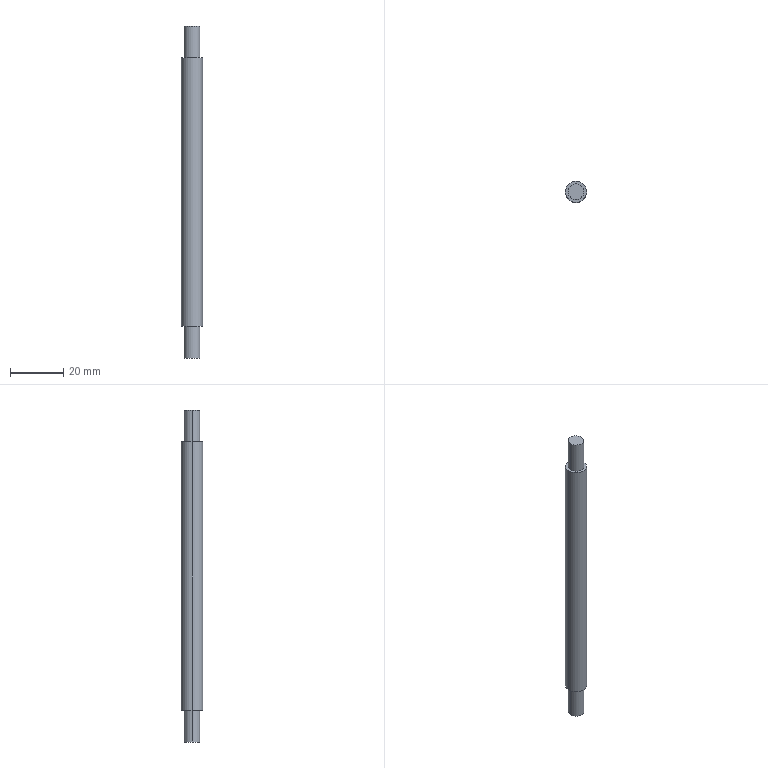Component | SolidWorks | TAR-02-024PaperPressWheelAxis-1 | 1 solid | 10 faces | box 8 x 8 x 125 mm | volume 5755 mm3 | cylinder 6 | plane 4 | commonest cylinder face diameters 6 x4 8 x2
build123d program:
from build123d import *

# Parameters (mm, degrees)
SKETCH1_R           = 3
BOSS_EXTRUDE1_DEPTH = 12
SKETCH2_R           = 4
BOSS_EXTRUDE2_DEPTH = 101


with BuildPart() as part:
    # Sketch1 → Boss-Extrude1 (new body)
    with BuildSketch(Plane.XY):
        Circle(SKETCH1_R)
    boss_extrude1 = extrude(amount=BOSS_EXTRUDE1_DEPTH)

    # Sketch2 → Boss-Extrude2 (add)
    with BuildSketch(Plane.XY.offset(12)):
        Circle(SKETCH2_R)
    extrude(amount=BOSS_EXTRUDE2_DEPTH)

    # Mirror1: Boss-Extrude1 across plane
    add(boss_extrude1.mirror(Plane(origin=(0, 0, 62.5), x_dir=(1, 0, 0), z_dir=(0, 0, -1))))


solid = part.part

# Placed as in the assembly
solid = solid.moved(Location((8.333, 43.101, -156.165), (0, 0, 0)))
STEP:
#1=CARTESIAN_POINT('',(0.4462,1.697,-1.699));
#2=VERTEX_POINT('',#1);
#3=CARTESIAN_POINT('',(0.2099,1.697,-1.699));
#4=VERTEX_POINT('',#3);
#5=CARTESIAN_POINT('',(0.3281,1.697,-1.699));
#6=DIRECTION('',(0.,0.,1.));
#7=DIRECTION('',(1.,0.,0.));
#8=AXIS2_PLACEMENT_3D('',#5,#6,#7);
#9=CIRCLE('',#8,0.1181);
#10=EDGE_CURVE('',#2,#4,#9,.T.);
#11=ORIENTED_EDGE('',*,*,#10,.T.);
#12=CARTESIAN_POINT('',(0.2099,1.697,-1.227));
#13=VERTEX_POINT('',#12);
#14=CARTESIAN_POINT('',(0.2099,1.697,-1.699));
#15=DIRECTION('',(0.,0.,1.));
#16=VECTOR('',#15,39.37);
#17=LINE('',#14,#16);
#18=EDGE_CURVE('',#4,#13,#17,.T.);
#19=ORIENTED_EDGE('',*,*,#18,.T.);
#20=CARTESIAN_POINT('',(0.4462,1.697,-1.227));
#21=VERTEX_POINT('',#20);
#22=CARTESIAN_POINT('',(0.3281,1.697,-1.227));
#23=DIRECTION('',(0.,0.,1.));
#24=DIRECTION('',(1.,0.,0.));
#25=AXIS2_PLACEMENT_3D('',#22,#23,#24);
#26=CIRCLE('',#25,0.1181);
#27=EDGE_CURVE('',#21,#13,#26,.T.);
#28=ORIENTED_EDGE('',*,*,#27,.F.);
#29=CARTESIAN_POINT('',(0.4462,1.697,-1.699));
#30=DIRECTION('',(0.,0.,1.));
#31=VECTOR('',#30,39.37);
#32=LINE('',#29,#31);
#33=EDGE_CURVE('',#2,#21,#32,.T.);
#34=ORIENTED_EDGE('',*,*,#33,.F.);
#35=EDGE_LOOP('',(#11,#19,#28,#34));
#36=FACE_OUTER_BOUND('',#35,.T.);
#37=CARTESIAN_POINT('',(0.3281,1.697,-1.699));
#38=DIRECTION('',(0.,0.,1.));
#39=DIRECTION('',(1.,0.,0.));
#40=AXIS2_PLACEMENT_3D('',#37,#38,#39);
#41=CYLINDRICAL_SURFACE('',#40,0.1181);
#42=ADVANCED_FACE('',(#36),#41,.T.);
#43=CARTESIAN_POINT('',(0.4855,1.697,-1.699));
#44=VERTEX_POINT('',#43);
#45=CARTESIAN_POINT('',(0.1706,1.697,-1.699));
#46=VERTEX_POINT('',#45);
#47=CARTESIAN_POINT('',(0.3281,1.697,-1.699));
#48=DIRECTION('',(0.,0.,1.));
#49=DIRECTION('',(1.,0.,0.));
#50=AXIS2_PLACEMENT_3D('',#47,#48,#49);
#51=CIRCLE('',#50,0.1575);
#52=EDGE_CURVE('',#44,#46,#51,.T.);
#53=ORIENTED_EDGE('',*,*,#52,.F.);
#54=CARTESIAN_POINT('',(0.4855,1.697,-5.676));
#55=VERTEX_POINT('',#54);
#56=CARTESIAN_POINT('',(0.4855,1.697,-1.699));
#57=DIRECTION('',(0.,0.,-1.));
#58=VECTOR('',#57,39.37);
#59=LINE('',#56,#58);
#60=EDGE_CURVE('',#44,#55,#59,.T.);
#61=ORIENTED_EDGE('',*,*,#60,.T.);
#62=CARTESIAN_POINT('',(0.1706,1.697,-5.676));
#63=VERTEX_POINT('',#62);
#64=CARTESIAN_POINT('',(0.3281,1.697,-5.676));
#65=DIRECTION('',(0.,0.,1.));
#66=DIRECTION('',(1.,0.,0.));
#67=AXIS2_PLACEMENT_3D('',#64,#65,#66);
#68=CIRCLE('',#67,0.1575);
#69=EDGE_CURVE('',#55,#63,#68,.T.);
#70=ORIENTED_EDGE('',*,*,#69,.T.);
#71=CARTESIAN_POINT('',(0.1706,1.697,-1.699));
#72=DIRECTION('',(0.,0.,-1.));
#73=VECTOR('',#72,39.37);
#74=LINE('',#71,#73);
#75=EDGE_CURVE('',#46,#63,#74,.T.);
#76=ORIENTED_EDGE('',*,*,#75,.F.);
#77=EDGE_LOOP('',(#53,#61,#70,#76));
#78=FACE_OUTER_BOUND('',#77,.T.);
#79=CARTESIAN_POINT('',(0.3281,1.697,-1.699));
#80=DIRECTION('',(0.,0.,-1.));
#81=DIRECTION('',(-1.,0.,0.));
#82=AXIS2_PLACEMENT_3D('',#79,#80,#81);
#83=CYLINDRICAL_SURFACE('',#82,0.1575);
#84=ADVANCED_FACE('',(#78),#83,.T.);
#85=CARTESIAN_POINT('',(0.4462,1.697,-5.676));
#86=VERTEX_POINT('',#85);
#87=CARTESIAN_POINT('',(0.2099,1.697,-5.676));
#88=VERTEX_POINT('',#87);
#89=CARTESIAN_POINT('',(0.3281,1.697,-5.676));
#90=DIRECTION('',(0.,0.,1.));
#91=DIRECTION('',(1.,0.,0.));
#92=AXIS2_PLACEMENT_3D('',#89,#90,#91);
#93=CIRCLE('',#92,0.1181);
#94=EDGE_CURVE('',#86,#88,#93,.T.);
#95=ORIENTED_EDGE('',*,*,#94,.F.);
#96=CARTESIAN_POINT('',(0.4462,1.697,-6.148));
#97=VERTEX_POINT('',#96);
#98=CARTESIAN_POINT('',(0.4462,1.697,-5.676));
#99=DIRECTION('',(0.,0.,-1.));
#100=VECTOR('',#99,39.37);
#101=LINE('',#98,#100);
#102=EDGE_CURVE('',#86,#97,#101,.T.);
#103=ORIENTED_EDGE('',*,*,#102,.T.);
#104=CARTESIAN_POINT('',(0.2099,1.697,-6.148));
#105=VERTEX_POINT('',#104);
#106=CARTESIAN_POINT('',(0.3281,1.697,-6.148));
#107=DIRECTION('',(0.,0.,1.));
#108=DIRECTION('',(1.,0.,0.));
#109=AXIS2_PLACEMENT_3D('',#106,#107,#108);
#110=CIRCLE('',#109,0.1181);
#111=EDGE_CURVE('',#97,#105,#110,.T.);
#112=ORIENTED_EDGE('',*,*,#111,.T.);
#113=CARTESIAN_POINT('',(0.2099,1.697,-5.676));
#114=DIRECTION('',(0.,0.,-1.));
#115=VECTOR('',#114,39.37);
#116=LINE('',#113,#115);
#117=EDGE_CURVE('',#88,#105,#116,.T.);
#118=ORIENTED_EDGE('',*,*,#117,.F.);
#119=EDGE_LOOP('',(#95,#103,#112,#118));
#120=FACE_OUTER_BOUND('',#119,.T.);
#121=CARTESIAN_POINT('',(0.3281,1.697,-5.676));
#122=DIRECTION('',(0.,0.,-1.));
#123=DIRECTION('',(-1.,0.,0.));
#124=AXIS2_PLACEMENT_3D('',#121,#122,#123);
#125=CYLINDRICAL_SURFACE('',#124,0.1181);
#126=ADVANCED_FACE('',(#120),#125,.T.);
#127=ORIENTED_EDGE('',*,*,#102,.F.);
#128=CARTESIAN_POINT('',(0.3281,1.697,-5.676));
#129=DIRECTION('',(0.,0.,1.));
#130=DIRECTION('',(1.,0.,0.));
#131=AXIS2_PLACEMENT_3D('',#128,#129,#130);
#132=CIRCLE('',#131,0.1181);
#133=EDGE_CURVE('',#88,#86,#132,.T.);
#134=ORIENTED_EDGE('',*,*,#133,.F.);
#135=ORIENTED_EDGE('',*,*,#117,.T.);
#136=CARTESIAN_POINT('',(0.3281,1.697,-6.148));
#137=DIRECTION('',(0.,0.,1.));
#138=DIRECTION('',(1.,0.,0.));
#139=AXIS2_PLACEMENT_3D('',#136,#137,#138);
#140=CIRCLE('',#139,0.1181);
#141=EDGE_CURVE('',#105,#97,#140,.T.);
#142=ORIENTED_EDGE('',*,*,#141,.T.);
#143=EDGE_LOOP('',(#127,#134,#135,#142));
#144=FACE_OUTER_BOUND('',#143,.T.);
#145=CARTESIAN_POINT('',(0.3281,1.697,-5.676));
#146=DIRECTION('',(0.,0.,-1.));
#147=DIRECTION('',(-1.,0.,0.));
#148=AXIS2_PLACEMENT_3D('',#145,#146,#147);
#149=CYLINDRICAL_SURFACE('',#148,0.1181);
#150=ADVANCED_FACE('',(#144),#149,.T.);
#151=ORIENTED_EDGE('',*,*,#141,.F.);
#152=ORIENTED_EDGE('',*,*,#111,.F.);
#153=EDGE_LOOP('',(#151,#152));
#154=FACE_OUTER_BOUND('',#153,.T.);
#155=CARTESIAN_POINT('',(0.3281,1.697,-6.148));
#156=DIRECTION('',(0.,0.,1.));
#157=DIRECTION('',(1.,0.,0.));
#158=AXIS2_PLACEMENT_3D('',#155,#156,#157);
#159=PLANE('',#158);
#160=ADVANCED_FACE('',(#154),#159,.F.);
#161=ORIENTED_EDGE('',*,*,#60,.F.);
#162=CARTESIAN_POINT('',(0.3281,1.697,-1.699));
#163=DIRECTION('',(0.,0.,1.));
#164=DIRECTION('',(1.,0.,0.));
#165=AXIS2_PLACEMENT_3D('',#162,#163,#164);
#166=CIRCLE('',#165,0.1575);
#167=EDGE_CURVE('',#46,#44,#166,.T.);
#168=ORIENTED_EDGE('',*,*,#167,.F.);
#169=ORIENTED_EDGE('',*,*,#75,.T.);
#170=CARTESIAN_POINT('',(0.3281,1.697,-5.676));
#171=DIRECTION('',(0.,0.,1.));
#172=DIRECTION('',(1.,0.,0.));
#173=AXIS2_PLACEMENT_3D('',#170,#171,#172);
#174=CIRCLE('',#173,0.1575);
#175=EDGE_CURVE('',#63,#55,#174,.T.);
#176=ORIENTED_EDGE('',*,*,#175,.T.);
#177=EDGE_LOOP('',(#161,#168,#169,#176));
#178=FACE_OUTER_BOUND('',#177,.T.);
#179=CARTESIAN_POINT('',(0.3281,1.697,-1.699));
#180=DIRECTION('',(0.,0.,-1.));
#181=DIRECTION('',(-1.,0.,0.));
#182=AXIS2_PLACEMENT_3D('',#179,#180,#181);
#183=CYLINDRICAL_SURFACE('',#182,0.1575);
#184=ADVANCED_FACE('',(#178),#183,.T.);
#185=ORIENTED_EDGE('',*,*,#10,.F.);
#186=CARTESIAN_POINT('',(0.3281,1.697,-1.699));
#187=DIRECTION('',(0.,0.,1.));
#188=DIRECTION('',(1.,0.,0.));
#189=AXIS2_PLACEMENT_3D('',#186,#187,#188);
#190=CIRCLE('',#189,0.1181);
#191=EDGE_CURVE('',#4,#2,#190,.T.);
#192=ORIENTED_EDGE('',*,*,#191,.F.);
#193=EDGE_LOOP('',(#185,#192));
#194=FACE_BOUND('',#193,.T.);
#195=ORIENTED_EDGE('',*,*,#167,.T.);
#196=ORIENTED_EDGE('',*,*,#52,.T.);
#197=EDGE_LOOP('',(#195,#196));
#198=FACE_OUTER_BOUND('',#197,.T.);
#199=CARTESIAN_POINT('',(0.3281,1.697,-1.699));
#200=DIRECTION('',(0.,0.,1.));
#201=DIRECTION('',(1.,0.,0.));
#202=AXIS2_PLACEMENT_3D('',#199,#200,#201);
#203=PLANE('',#202);
#204=ADVANCED_FACE('',(#194,#198),#203,.T.);
#205=ORIENTED_EDGE('',*,*,#133,.T.);
#206=ORIENTED_EDGE('',*,*,#94,.T.);
#207=EDGE_LOOP('',(#205,#206));
#208=FACE_BOUND('',#207,.T.);
#209=ORIENTED_EDGE('',*,*,#175,.F.);
#210=ORIENTED_EDGE('',*,*,#69,.F.);
#211=EDGE_LOOP('',(#209,#210));
#212=FACE_OUTER_BOUND('',#211,.T.);
#213=CARTESIAN_POINT('',(0.3281,1.697,-5.676));
#214=DIRECTION('',(0.,0.,1.));
#215=DIRECTION('',(1.,0.,0.));
#216=AXIS2_PLACEMENT_3D('',#213,#214,#215);
#217=PLANE('',#216);
#218=ADVANCED_FACE('',(#208,#212),#217,.F.);
#219=ORIENTED_EDGE('',*,*,#18,.F.);
#220=ORIENTED_EDGE('',*,*,#191,.T.);
#221=ORIENTED_EDGE('',*,*,#33,.T.);
#222=CARTESIAN_POINT('',(0.3281,1.697,-1.227));
#223=DIRECTION('',(0.,0.,1.));
#224=DIRECTION('',(1.,0.,0.));
#225=AXIS2_PLACEMENT_3D('',#222,#223,#224);
#226=CIRCLE('',#225,0.1181);
#227=EDGE_CURVE('',#13,#21,#226,.T.);
#228=ORIENTED_EDGE('',*,*,#227,.F.);
#229=EDGE_LOOP('',(#219,#220,#221,#228));
#230=FACE_OUTER_BOUND('',#229,.T.);
#231=CARTESIAN_POINT('',(0.3281,1.697,-1.699));
#232=DIRECTION('',(0.,0.,1.));
#233=DIRECTION('',(1.,0.,0.));
#234=AXIS2_PLACEMENT_3D('',#231,#232,#233);
#235=CYLINDRICAL_SURFACE('',#234,0.1181);
#236=ADVANCED_FACE('',(#230),#235,.T.);
#237=ORIENTED_EDGE('',*,*,#27,.T.);
#238=ORIENTED_EDGE('',*,*,#227,.T.);
#239=EDGE_LOOP('',(#237,#238));
#240=FACE_OUTER_BOUND('',#239,.T.);
#241=CARTESIAN_POINT('',(0.3281,1.697,-1.227));
#242=DIRECTION('',(0.,0.,-1.));
#243=DIRECTION('',(1.,0.,0.));
#244=AXIS2_PLACEMENT_3D('',#241,#242,#243);
#245=PLANE('',#244);
#246=ADVANCED_FACE('',(#240),#245,.F.);
#247=CLOSED_SHELL('',(#42,#84,#126,#150,#160,#184,#204,#218,#236,#246));
#248=MANIFOLD_SOLID_BREP('',#247);
#249=CARTESIAN_POINT('',(0.,0.,0.));
#250=DIRECTION('',(0.,0.,1.));
#251=DIRECTION('',(1.,0.,0.));
#252=AXIS2_PLACEMENT_3D('',#249,#250,#251);
#253=(LENGTH_UNIT()NAMED_UNIT(*)SI_UNIT($,.METRE.));
#254=LENGTH_MEASURE_WITH_UNIT(LENGTH_MEASURE(0.0254),#253);
#255=DIMENSIONAL_EXPONENTS(1.,0.,0.,0.,0.,0.,0.);
#256=(CONVERSION_BASED_UNIT('',#254)LENGTH_UNIT()NAMED_UNIT(#255));
#257=UNCERTAINTY_MEASURE_WITH_UNIT(LENGTH_MEASURE(0.00001),#256,'','');
#258=(NAMED_UNIT(*)PLANE_ANGLE_UNIT()SI_UNIT($,.RADIAN.));
#259=(NAMED_UNIT(*)SI_UNIT($,.STERADIAN.)SOLID_ANGLE_UNIT());
#260=(GEOMETRIC_REPRESENTATION_CONTEXT(3)GLOBAL_UNCERTAINTY_ASSIGNED_CONTEXT((#257))GLOBAL_UNIT_ASSIGNED_CONTEXT((#256,#258,#259))REPRESENTATION_CONTEXT('',''));
#261=ADVANCED_BREP_SHAPE_REPRESENTATION('',(#248,#252),#260);
#262=COLOUR_RGB('',0.7922,0.8196,0.9333);
#263=FILL_AREA_STYLE_COLOUR('',#262);
#264=FILL_AREA_STYLE('',(#263));
#265=SURFACE_STYLE_FILL_AREA(#264);
#266=SURFACE_SIDE_STYLE('',(#265));
#267=SURFACE_STYLE_USAGE(.BOTH.,#266);
#268=PRESENTATION_STYLE_ASSIGNMENT((#267));
#269=STYLED_ITEM('',(#268),#248);
#270=PRESENTATION_LAYER_ASSIGNMENT('','',(#269));
#271=(LENGTH_UNIT()NAMED_UNIT(*)SI_UNIT($,.METRE.));
#272=LENGTH_MEASURE_WITH_UNIT(LENGTH_MEASURE(0.0254),#271);
#273=DIMENSIONAL_EXPONENTS(1.,0.,0.,0.,0.,0.,0.);
#274=(CONVERSION_BASED_UNIT('',#272)LENGTH_UNIT()NAMED_UNIT(#273));
#275=UNCERTAINTY_MEASURE_WITH_UNIT(LENGTH_MEASURE(0.00001),#274,'','');
#276=(NAMED_UNIT(*)PLANE_ANGLE_UNIT()SI_UNIT($,.RADIAN.));
#277=(NAMED_UNIT(*)SI_UNIT($,.STERADIAN.)SOLID_ANGLE_UNIT());
#278=(GEOMETRIC_REPRESENTATION_CONTEXT(3)GLOBAL_UNCERTAINTY_ASSIGNED_CONTEXT((#275))GLOBAL_UNIT_ASSIGNED_CONTEXT((#274,#276,#277))REPRESENTATION_CONTEXT('',''));
#279=MECHANICAL_DESIGN_GEOMETRIC_PRESENTATION_REPRESENTATION('',(#269),#278);